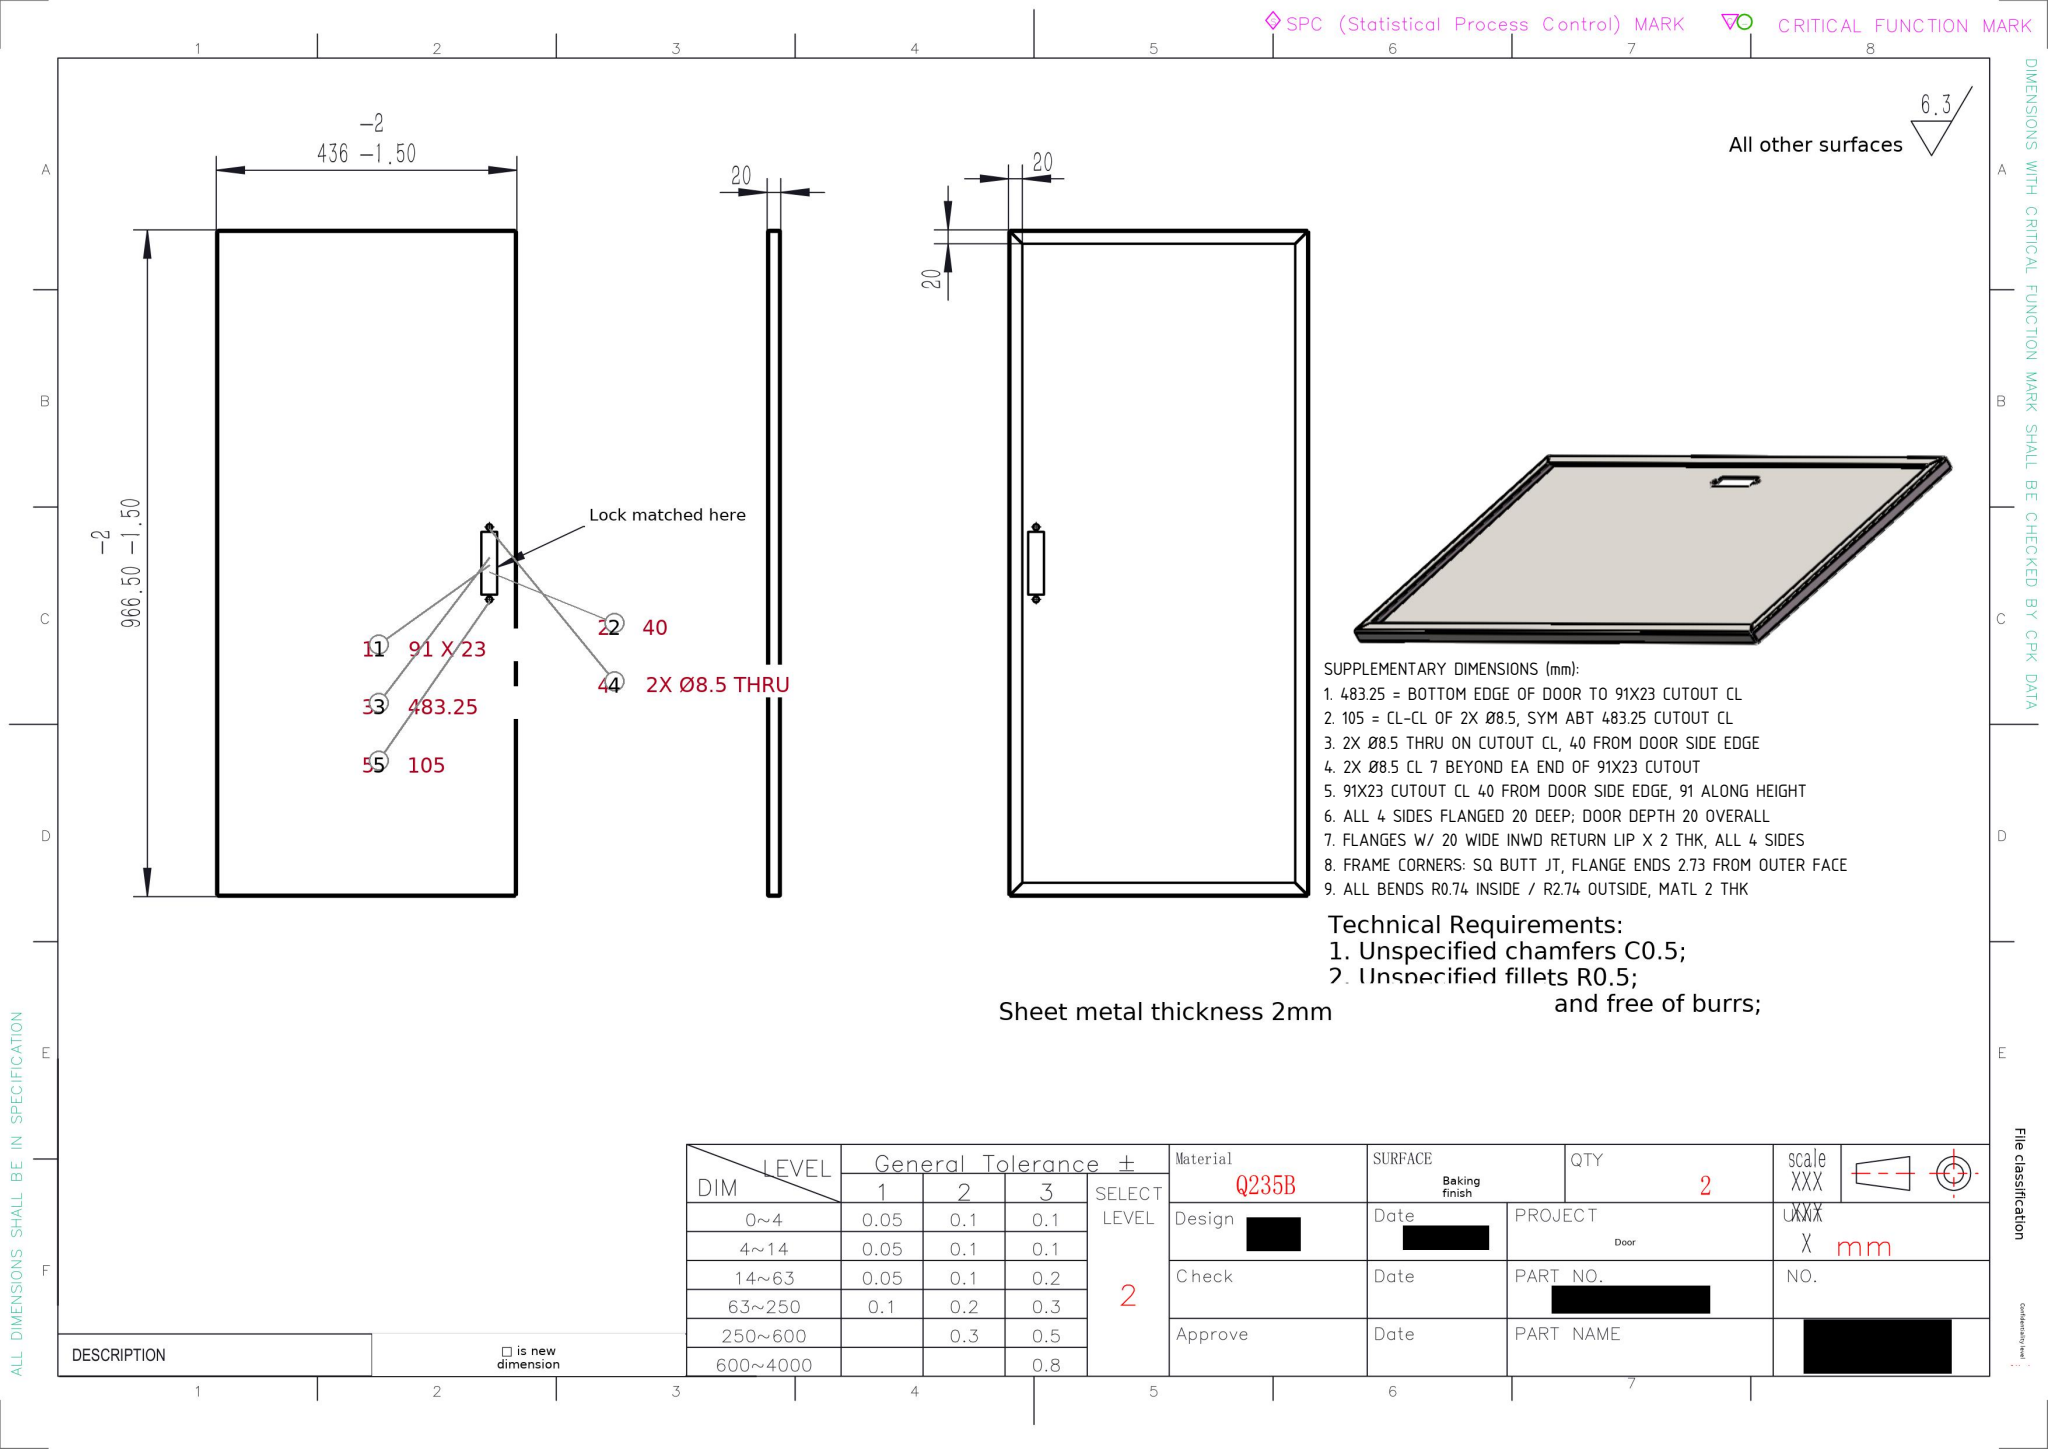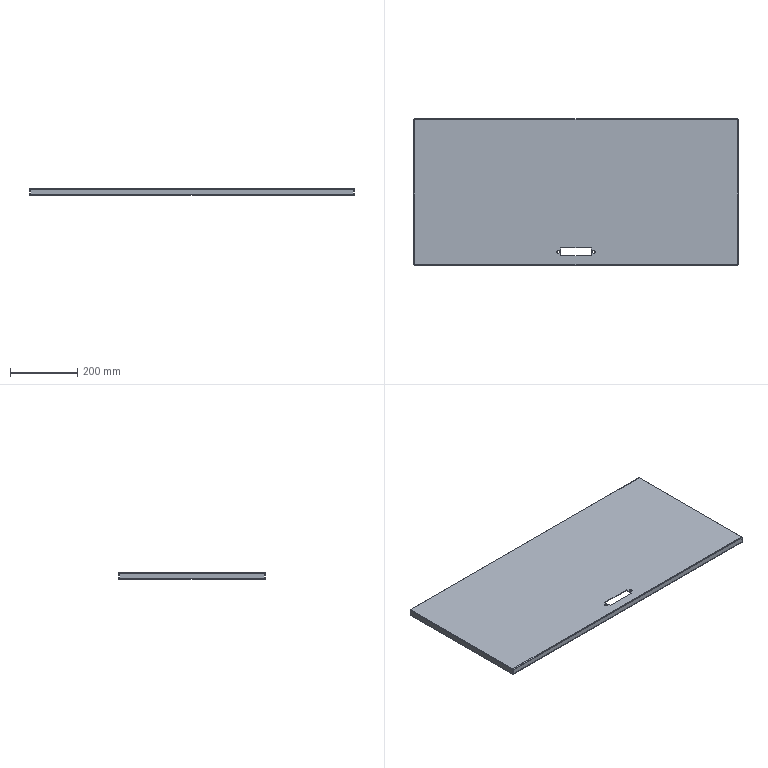Part | SolidWorks | mm | 1 solid | 78 faces | box 966.5 x 436 x 20 mm | volume 1027814 mm3 | plane 42 | cylinder 20 | spline 16 | commonest cylinder face diameters 5.473 x8 1.473 x8 8.5 x4